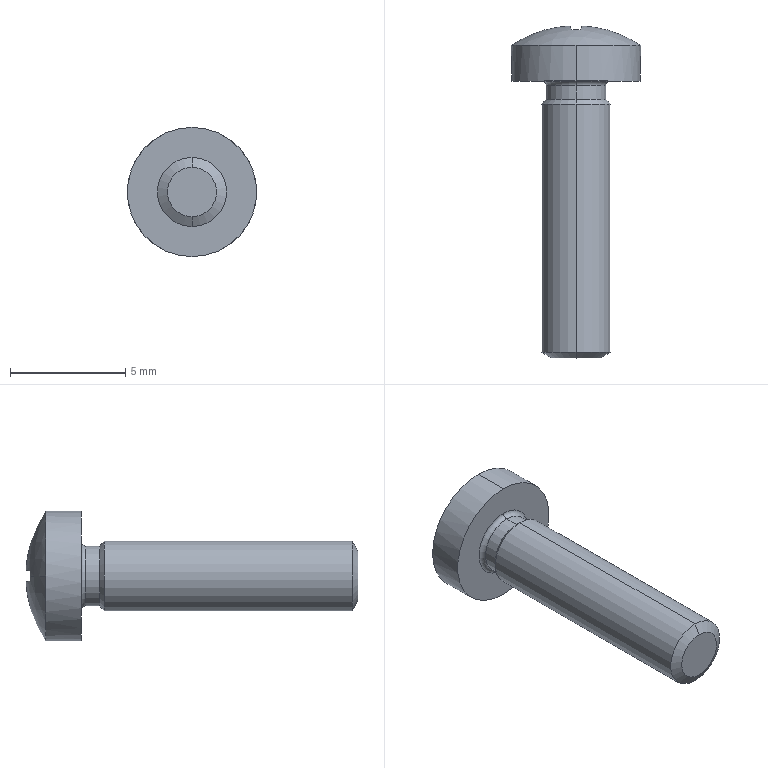Component | SolidWorks | GB_T818-2000PhillipsPanHeadScrewM3_12-3 | 1 solid | 28 faces | box 5.6 x 14.39 x 5.6 mm | volume 130 mm3 | plane 14 | cylinder 6 | cone 4 | torus 2 | sphere 2 | commonest cylinder face diameters 2.598 x2 5.6 x2 3 x2
build123d program:
from build123d import *


with BuildPart() as part:
    # Sketch2 → Base-Revolve (revolve)
    with BuildSketch(Plane.XY, mode=Mode.PRIVATE) as base_revolve_sk:
        with BuildLine():
            Line((0, 0), (14.4, 0))
            Line((14.4, 0), (14.4, 1.5))
            Line((14.4, 1.5), (3.4, 1.5))
            Line((3.4, 1.5), (3.199, 1.299))
            Line((3.199, 1.299), (2.601, 1.299))
            ThreePointArc((2.601, 1.299), (2.459, 1.358), (2.4, 1.5))
            Line((2.4, 1.5), (2.4, 2.8))
            Line((2.4, 2.8), (0.8575, 2.8))
            ThreePointArc((0.8575, 2.8), (0.2192, 1.464), (0, 0))
        make_face()
    revolve(base_revolve_sk.sketch.rotate(Axis((-1.332, 0, 0), (1, 0, 0)), 90), axis=Axis((-1.332, 0, 0), (1, 0, 0)))

    # Sketch3 → Cut-Revolve1 (revolve, cut)
    with BuildSketch(Plane.XY, mode=Mode.PRIVATE) as cut_revolve1_sk:
        Polygon((14.153, 1.5), (14.653, 1.5), (14.4, 1.067), align=None)
    revolve(cut_revolve1_sk.sketch.rotate(Axis((-0.2428, 0, 0), (1, 0, 0)), 90), axis=Axis((-0.2428, 0, 0), (1, 0, 0)), mode=Mode.SUBTRACT)

    # Sketch5 → Cut-Loft1 section 0
    with BuildSketch(Plane(origin=(0, 0, 0), x_dir=(0, 0, -1), z_dir=(1, 0, 0)), mode=Mode.PRIVATE) as cut_loft1_s0:
        with BuildLine():
            Line((0.25, 1.5), (-0.25, 1.5))
            Line((-0.25, 1.5), (-0.25, -1.5))
            Line((-0.25, -1.5), (0.25, -1.5))
            Line((0.25, -1.5), (0.25, 1.5))
        make_face()
    cut_loft1 = loft([Vertex(1.8, 0, 0), cut_loft1_s0.sketch], mode=Mode.SUBTRACT)

    # Mirror1: Cut-Loft1 across plane
    add(cut_loft1.mirror(Plane(origin=(0, 0, 0), x_dir=(0, 0.7071, 0.7071), z_dir=(0, -0.7071, 0.7071))), mode=Mode.SUBTRACT)


solid = part.part

# Placed as in the assembly
solid = solid.moved(Location((-27.344, 162.966, -166.507), (0, 0, -90)))
STEP:
#1=COLOUR_RGB('',0.7922,0.8196,0.9333);
#2=FILL_AREA_STYLE_COLOUR('',#1);
#3=FILL_AREA_STYLE('',(#2));
#4=SURFACE_STYLE_FILL_AREA(#3);
#5=SURFACE_SIDE_STYLE('',(#4));
#6=SURFACE_STYLE_USAGE(.BOTH.,#5);
#7=PRESENTATION_STYLE_ASSIGNMENT((#6));
#8=CARTESIAN_POINT('',(-1.077,5.849,-6.513));
#9=VERTEX_POINT('',#8);
#10=CARTESIAN_POINT('',(-1.077,5.849,-6.597));
#11=VERTEX_POINT('',#10);
#12=CARTESIAN_POINT('',(-1.077,5.849,-6.555));
#13=DIRECTION('',(0.,1.,0.));
#14=DIRECTION('',(0.,0.,1.));
#15=AXIS2_PLACEMENT_3D('',#12,#13,#14);
#16=CIRCLE('',#15,0.04201);
#17=EDGE_CURVE('',#9,#11,#16,.T.);
#18=ORIENTED_EDGE('',*,*,#17,.T.);
#19=CARTESIAN_POINT('',(-1.077,5.859,-6.614));
#20=VERTEX_POINT('',#19);
#21=CARTESIAN_POINT('',(-1.077,5.859,-6.614));
#22=DIRECTION('',(0.,0.4959,-0.8684));
#23=VECTOR('',#22,39.37);
#24=LINE('',#21,#23);
#25=EDGE_CURVE('',#11,#20,#24,.T.);
#26=ORIENTED_EDGE('',*,*,#25,.T.);
#27=CARTESIAN_POINT('',(-1.077,5.859,-6.496));
#28=VERTEX_POINT('',#27);
#29=CARTESIAN_POINT('',(-1.077,5.859,-6.555));
#30=DIRECTION('',(0.,1.,0.));
#31=DIRECTION('',(0.,0.,1.));
#32=AXIS2_PLACEMENT_3D('',#29,#30,#31);
#33=CIRCLE('',#32,0.05906);
#34=EDGE_CURVE('',#28,#20,#33,.T.);
#35=ORIENTED_EDGE('',*,*,#34,.F.);
#36=CARTESIAN_POINT('',(-1.077,5.859,-6.496));
#37=DIRECTION('',(0.,0.4959,0.8684));
#38=VECTOR('',#37,39.37);
#39=LINE('',#36,#38);
#40=EDGE_CURVE('',#9,#28,#39,.T.);
#41=ORIENTED_EDGE('',*,*,#40,.F.);
#42=EDGE_LOOP('',(#18,#26,#35,#41));
#43=FACE_OUTER_BOUND('',#42,.T.);
#44=CARTESIAN_POINT('',(-1.077,5.859,-6.555));
#45=DIRECTION('',(0.,1.,0.));
#46=DIRECTION('',(0.,0.,1.));
#47=AXIS2_PLACEMENT_3D('',#44,#45,#46);
#48=CONICAL_SURFACE('',#47,0.05906,1.052);
#49=ADVANCED_FACE('',(#43),#48,.T.);
#50=CARTESIAN_POINT('',(-1.077,6.29,-6.504));
#51=VERTEX_POINT('',#50);
#52=CARTESIAN_POINT('',(-1.077,6.29,-6.607));
#53=VERTEX_POINT('',#52);
#54=CARTESIAN_POINT('',(-1.077,6.29,-6.555));
#55=DIRECTION('',(0.,1.,0.));
#56=DIRECTION('',(0.,0.,1.));
#57=AXIS2_PLACEMENT_3D('',#54,#55,#56);
#58=CIRCLE('',#57,0.05114);
#59=EDGE_CURVE('',#51,#53,#58,.T.);
#60=ORIENTED_EDGE('',*,*,#59,.F.);
#61=CARTESIAN_POINT('',(-1.077,6.282,-6.496));
#62=VERTEX_POINT('',#61);
#63=CARTESIAN_POINT('',(-1.077,6.282,-6.496));
#64=DIRECTION('',(0.,-0.7071,0.7071));
#65=VECTOR('',#64,39.37);
#66=LINE('',#63,#65);
#67=EDGE_CURVE('',#51,#62,#66,.T.);
#68=ORIENTED_EDGE('',*,*,#67,.T.);
#69=CARTESIAN_POINT('',(-1.077,6.282,-6.614));
#70=VERTEX_POINT('',#69);
#71=CARTESIAN_POINT('',(-1.077,6.282,-6.555));
#72=DIRECTION('',(0.,1.,0.));
#73=DIRECTION('',(0.,0.,1.));
#74=AXIS2_PLACEMENT_3D('',#71,#72,#73);
#75=CIRCLE('',#74,0.05906);
#76=EDGE_CURVE('',#62,#70,#75,.T.);
#77=ORIENTED_EDGE('',*,*,#76,.T.);
#78=CARTESIAN_POINT('',(-1.077,6.282,-6.614));
#79=DIRECTION('',(0.,-0.7071,-0.7071));
#80=VECTOR('',#79,39.37);
#81=LINE('',#78,#80);
#82=EDGE_CURVE('',#53,#70,#81,.T.);
#83=ORIENTED_EDGE('',*,*,#82,.F.);
#84=EDGE_LOOP('',(#60,#68,#77,#83));
#85=FACE_OUTER_BOUND('',#84,.T.);
#86=CARTESIAN_POINT('',(-1.077,6.282,-6.555));
#87=DIRECTION('',(0.,-1.,0.));
#88=DIRECTION('',(0.,0.,-1.));
#89=AXIS2_PLACEMENT_3D('',#86,#87,#88);
#90=CONICAL_SURFACE('',#89,0.05906,0.7854);
#91=ADVANCED_FACE('',(#85),#90,.T.);
#92=ORIENTED_EDGE('',*,*,#59,.T.);
#93=CARTESIAN_POINT('',(-1.077,6.314,-6.607));
#94=VERTEX_POINT('',#93);
#95=CARTESIAN_POINT('',(-1.077,6.468,-6.607));
#96=DIRECTION('',(0.,1.,0.));
#97=VECTOR('',#96,39.37);
#98=LINE('',#95,#97);
#99=EDGE_CURVE('',#53,#94,#98,.T.);
#100=ORIENTED_EDGE('',*,*,#99,.T.);
#101=CARTESIAN_POINT('',(-1.077,6.314,-6.504));
#102=VERTEX_POINT('',#101);
#103=CARTESIAN_POINT('',(-1.077,6.314,-6.555));
#104=DIRECTION('',(0.,1.,0.));
#105=DIRECTION('',(0.,0.,1.));
#106=AXIS2_PLACEMENT_3D('',#103,#104,#105);
#107=CIRCLE('',#106,0.05114);
#108=EDGE_CURVE('',#102,#94,#107,.T.);
#109=ORIENTED_EDGE('',*,*,#108,.F.);
#110=CARTESIAN_POINT('',(-1.077,6.468,-6.504));
#111=DIRECTION('',(0.,1.,0.));
#112=VECTOR('',#111,39.37);
#113=LINE('',#110,#112);
#114=EDGE_CURVE('',#51,#102,#113,.T.);
#115=ORIENTED_EDGE('',*,*,#114,.F.);
#116=EDGE_LOOP('',(#92,#100,#109,#115));
#117=FACE_OUTER_BOUND('',#116,.T.);
#118=CARTESIAN_POINT('',(-1.077,6.468,-6.555));
#119=DIRECTION('',(0.,1.,0.));
#120=DIRECTION('',(0.,0.,1.));
#121=AXIS2_PLACEMENT_3D('',#118,#119,#120);
#122=CYLINDRICAL_SURFACE('',#121,0.05114);
#123=ADVANCED_FACE('',(#117),#122,.T.);
#124=CARTESIAN_POINT('',(-1.077,6.321,-6.614));
#125=VERTEX_POINT('',#124);
#126=CARTESIAN_POINT('',(-1.077,6.321,-6.496));
#127=VERTEX_POINT('',#126);
#128=CARTESIAN_POINT('',(-1.077,6.321,-6.555));
#129=DIRECTION('',(0.,1.,0.));
#130=DIRECTION('',(0.,0.,1.));
#131=AXIS2_PLACEMENT_3D('',#128,#129,#130);
#132=CIRCLE('',#131,0.05906);
#133=EDGE_CURVE('',#125,#127,#132,.T.);
#134=ORIENTED_EDGE('',*,*,#133,.F.);
#135=CARTESIAN_POINT('',(-1.077,6.314,-6.614));
#136=DIRECTION('',(1.,0.,0.));
#137=DIRECTION('',(0.,0.,-1.));
#138=AXIS2_PLACEMENT_3D('',#135,#136,#137);
#139=CIRCLE('',#138,0.007913);
#140=EDGE_CURVE('',#125,#94,#139,.T.);
#141=ORIENTED_EDGE('',*,*,#140,.T.);
#142=CARTESIAN_POINT('',(-1.077,6.314,-6.555));
#143=DIRECTION('',(0.,1.,0.));
#144=DIRECTION('',(0.,0.,1.));
#145=AXIS2_PLACEMENT_3D('',#142,#143,#144);
#146=CIRCLE('',#145,0.05114);
#147=EDGE_CURVE('',#94,#102,#146,.T.);
#148=ORIENTED_EDGE('',*,*,#147,.T.);
#149=CARTESIAN_POINT('',(-1.077,6.314,-6.496));
#150=DIRECTION('',(-1.,0.,0.));
#151=DIRECTION('',(0.,0.,1.));
#152=AXIS2_PLACEMENT_3D('',#149,#150,#151);
#153=CIRCLE('',#152,0.007913);
#154=EDGE_CURVE('',#127,#102,#153,.T.);
#155=ORIENTED_EDGE('',*,*,#154,.F.);
#156=EDGE_LOOP('',(#134,#141,#148,#155));
#157=FACE_OUTER_BOUND('',#156,.T.);
#158=CARTESIAN_POINT('',(-1.077,6.314,-6.555));
#159=DIRECTION('',(0.,1.,0.));
#160=DIRECTION('',(0.,0.,1.));
#161=AXIS2_PLACEMENT_3D('',#158,#159,#160);
#162=TOROIDAL_SURFACE('',#161,0.05906,0.007913);
#163=ADVANCED_FACE('',(#157),#162,.F.);
#164=CARTESIAN_POINT('',(-1.077,6.321,-6.445));
#165=VERTEX_POINT('',#164);
#166=CARTESIAN_POINT('',(-1.077,6.321,-6.666));
#167=VERTEX_POINT('',#166);
#168=CARTESIAN_POINT('',(-1.077,6.321,-6.555));
#169=DIRECTION('',(0.,1.,0.));
#170=DIRECTION('',(0.,0.,1.));
#171=AXIS2_PLACEMENT_3D('',#168,#169,#170);
#172=CIRCLE('',#171,0.1102);
#173=EDGE_CURVE('',#165,#167,#172,.T.);
#174=ORIENTED_EDGE('',*,*,#173,.T.);
#175=CARTESIAN_POINT('',(-1.077,6.382,-6.666));
#176=VERTEX_POINT('',#175);
#177=CARTESIAN_POINT('',(-1.077,6.468,-6.666));
#178=DIRECTION('',(0.,1.,0.));
#179=VECTOR('',#178,39.37);
#180=LINE('',#177,#179);
#181=EDGE_CURVE('',#167,#176,#180,.T.);
#182=ORIENTED_EDGE('',*,*,#181,.T.);
#183=CARTESIAN_POINT('',(-0.9663,6.382,-6.555));
#184=VERTEX_POINT('',#183);
#185=CARTESIAN_POINT('',(-1.077,6.382,-6.555));
#186=DIRECTION('',(0.,1.,0.));
#187=DIRECTION('',(0.,0.,1.));
#188=AXIS2_PLACEMENT_3D('',#185,#186,#187);
#189=CIRCLE('',#188,0.1102);
#190=EDGE_CURVE('',#184,#176,#189,.T.);
#191=ORIENTED_EDGE('',*,*,#190,.F.);
#192=CARTESIAN_POINT('',(-1.077,6.382,-6.445));
#193=VERTEX_POINT('',#192);
#194=CARTESIAN_POINT('',(-1.077,6.382,-6.555));
#195=DIRECTION('',(0.,1.,0.));
#196=DIRECTION('',(0.,0.,1.));
#197=AXIS2_PLACEMENT_3D('',#194,#195,#196);
#198=CIRCLE('',#197,0.1102);
#199=EDGE_CURVE('',#193,#184,#198,.T.);
#200=ORIENTED_EDGE('',*,*,#199,.F.);
#201=CARTESIAN_POINT('',(-1.077,6.468,-6.445));
#202=DIRECTION('',(0.,1.,0.));
#203=VECTOR('',#202,39.37);
#204=LINE('',#201,#203);
#205=EDGE_CURVE('',#165,#193,#204,.T.);
#206=ORIENTED_EDGE('',*,*,#205,.F.);
#207=EDGE_LOOP('',(#174,#182,#191,#200,#206));
#208=FACE_OUTER_BOUND('',#207,.T.);
#209=CARTESIAN_POINT('',(-1.077,6.468,-6.555));
#210=DIRECTION('',(0.,1.,0.));
#211=DIRECTION('',(0.,0.,1.));
#212=AXIS2_PLACEMENT_3D('',#209,#210,#211);
#213=CYLINDRICAL_SURFACE('',#212,0.1102);
#214=ADVANCED_FACE('',(#208),#213,.T.);
#215=ORIENTED_EDGE('',*,*,#190,.T.);
#216=CARTESIAN_POINT('',(-1.187,6.382,-6.555));
#217=VERTEX_POINT('',#216);
#218=CARTESIAN_POINT('',(-1.077,6.382,-6.555));
#219=DIRECTION('',(0.,1.,0.));
#220=DIRECTION('',(0.,0.,1.));
#221=AXIS2_PLACEMENT_3D('',#218,#219,#220);
#222=CIRCLE('',#221,0.1102);
#223=EDGE_CURVE('',#176,#217,#222,.T.);
#224=ORIENTED_EDGE('',*,*,#223,.T.);
#225=CARTESIAN_POINT('',(-1.13,6.409,-6.555));
#226=VERTEX_POINT('',#225);
#227=CARTESIAN_POINT('',(-1.077,6.219,-6.555));
#228=DIRECTION('',(0.,0.,-1.));
#229=DIRECTION('',(-1.,0.,0.));
#230=AXIS2_PLACEMENT_3D('',#227,#228,#229);
#231=CIRCLE('',#230,0.1969);
#232=EDGE_CURVE('',#217,#226,#231,.T.);
#233=ORIENTED_EDGE('',*,*,#232,.T.);
#234=CARTESIAN_POINT('',(-1.129,6.409,-6.564));
#235=VERTEX_POINT('',#234);
#236=CARTESIAN_POINT('',(-1.015,6.271,-6.555));
#237=DIRECTION('',(-0.7682,-0.6402,0.));
#238=DIRECTION('',(0.6402,-0.7682,0.));
#239=AXIS2_PLACEMENT_3D('',#236,#237,#238);
#240=CIRCLE('',#239,0.1796);
#241=EDGE_CURVE('',#226,#235,#240,.T.);
#242=ORIENTED_EDGE('',*,*,#241,.T.);
#243=CARTESIAN_POINT('',(-1.086,6.415,-6.565));
#244=VERTEX_POINT('',#243);
#245=CARTESIAN_POINT('',(-1.077,6.222,-6.538));
#246=DIRECTION('',(0.,-0.1376,-0.9905));
#247=DIRECTION('',(0.,0.9905,-0.1376));
#248=AXIS2_PLACEMENT_3D('',#245,#246,#247);
#249=CIRCLE('',#248,0.1961);
#250=EDGE_CURVE('',#235,#244,#249,.T.);
#251=ORIENTED_EDGE('',*,*,#250,.T.);
#252=CARTESIAN_POINT('',(-1.085,6.409,-6.608));
#253=VERTEX_POINT('',#252);
#254=CARTESIAN_POINT('',(-1.059,6.222,-6.555));
#255=DIRECTION('',(-0.9905,-0.1376,-0.));
#256=DIRECTION('',(0.1376,-0.9905,0.));
#257=AXIS2_PLACEMENT_3D('',#254,#255,#256);
#258=CIRCLE('',#257,0.1961);
#259=EDGE_CURVE('',#244,#253,#258,.T.);
#260=ORIENTED_EDGE('',*,*,#259,.T.);
#261=CARTESIAN_POINT('',(-1.068,6.409,-6.608));
#262=VERTEX_POINT('',#261);
#263=CARTESIAN_POINT('',(-1.077,6.271,-6.493));
#264=DIRECTION('',(0.,-0.6402,-0.7682));
#265=DIRECTION('',(0.,0.7682,-0.6402));
#266=AXIS2_PLACEMENT_3D('',#263,#264,#265);
#267=CIRCLE('',#266,0.1796);
#268=EDGE_CURVE('',#253,#262,#267,.T.);
#269=ORIENTED_EDGE('',*,*,#268,.T.);
#270=CARTESIAN_POINT('',(-1.067,6.415,-6.565));
#271=VERTEX_POINT('',#270);
#272=CARTESIAN_POINT('',(-1.094,6.222,-6.555));
#273=DIRECTION('',(0.9905,-0.1376,0.));
#274=DIRECTION('',(0.1376,0.9905,0.));
#275=AXIS2_PLACEMENT_3D('',#272,#273,#274);
#276=CIRCLE('',#275,0.1961);
#277=EDGE_CURVE('',#262,#271,#276,.T.);
#278=ORIENTED_EDGE('',*,*,#277,.T.);
#279=CARTESIAN_POINT('',(-1.024,6.409,-6.564));
#280=VERTEX_POINT('',#279);
#281=CARTESIAN_POINT('',(-1.077,6.222,-6.538));
#282=DIRECTION('',(0.,-0.1376,-0.9905));
#283=DIRECTION('',(0.,0.9905,-0.1376));
#284=AXIS2_PLACEMENT_3D('',#281,#282,#283);
#285=CIRCLE('',#284,0.1961);
#286=EDGE_CURVE('',#271,#280,#285,.T.);
#287=ORIENTED_EDGE('',*,*,#286,.T.);
#288=CARTESIAN_POINT('',(-1.024,6.409,-6.555));
#289=VERTEX_POINT('',#288);
#290=CARTESIAN_POINT('',(-1.139,6.271,-6.555));
#291=DIRECTION('',(0.7682,-0.6402,0.));
#292=DIRECTION('',(0.6402,0.7682,0.));
#293=AXIS2_PLACEMENT_3D('',#290,#291,#292);
#294=CIRCLE('',#293,0.1796);
#295=EDGE_CURVE('',#280,#289,#294,.T.);
#296=ORIENTED_EDGE('',*,*,#295,.T.);
#297=CARTESIAN_POINT('',(-1.077,6.219,-6.555));
#298=DIRECTION('',(0.,0.,1.));
#299=DIRECTION('',(1.,0.,0.));
#300=AXIS2_PLACEMENT_3D('',#297,#298,#299);
#301=CIRCLE('',#300,0.1969);
#302=EDGE_CURVE('',#184,#289,#301,.T.);
#303=ORIENTED_EDGE('',*,*,#302,.F.);
#304=EDGE_LOOP('',(#215,#224,#233,#242,#251,#260,#269,#278,#287,#296,#303));
#305=FACE_OUTER_BOUND('',#304,.T.);
#306=CARTESIAN_POINT('',(-1.077,6.219,-6.555));
#307=DIRECTION('',(0.,0.,-1.));
#308=DIRECTION('',(1.,0.,0.));
#309=AXIS2_PLACEMENT_3D('',#306,#307,#308);
#310=SPHERICAL_SURFACE('',#309,0.1969);
#311=ADVANCED_FACE('',(#305),#310,.T.);
#312=ORIENTED_EDGE('',*,*,#34,.T.);
#313=CARTESIAN_POINT('',(-1.077,6.468,-6.614));
#314=DIRECTION('',(0.,1.,0.));
#315=VECTOR('',#314,39.37);
#316=LINE('',#313,#315);
#317=EDGE_CURVE('',#20,#70,#316,.T.);
#318=ORIENTED_EDGE('',*,*,#317,.T.);
#319=ORIENTED_EDGE('',*,*,#76,.F.);
#320=CARTESIAN_POINT('',(-1.077,6.468,-6.496));
#321=DIRECTION('',(0.,1.,0.));
#322=VECTOR('',#321,39.37);
#323=LINE('',#320,#322);
#324=EDGE_CURVE('',#28,#62,#323,.T.);
#325=ORIENTED_EDGE('',*,*,#324,.F.);
#326=EDGE_LOOP('',(#312,#318,#319,#325));
#327=FACE_OUTER_BOUND('',#326,.T.);
#328=CARTESIAN_POINT('',(-1.077,6.468,-6.555));
#329=DIRECTION('',(0.,1.,0.));
#330=DIRECTION('',(0.,0.,1.));
#331=AXIS2_PLACEMENT_3D('',#328,#329,#330);
#332=CYLINDRICAL_SURFACE('',#331,0.05906);
#333=ADVANCED_FACE('',(#327),#332,.T.);
#334=CARTESIAN_POINT('',(-1.077,6.345,-6.555));
#335=VERTEX_POINT('',#334);
#336=CARTESIAN_POINT('',(-1.077,6.345,-6.555));
#337=DIRECTION('',(-0.6366,0.7639,-0.1061));
#338=VECTOR('',#337,39.37);
#339=LINE('',#336,#338);
#340=EDGE_CURVE('',#335,#235,#339,.T.);
#341=ORIENTED_EDGE('',*,*,#340,.F.);
#342=CARTESIAN_POINT('',(-1.077,6.345,-6.555));
#343=DIRECTION('',(-0.1363,0.9813,-0.1363));
#344=VECTOR('',#343,39.37);
#345=LINE('',#342,#344);
#346=EDGE_CURVE('',#335,#244,#345,.T.);
#347=ORIENTED_EDGE('',*,*,#346,.T.);
#348=ORIENTED_EDGE('',*,*,#250,.F.);
#349=EDGE_LOOP('',(#341,#347,#348));
#350=FACE_OUTER_BOUND('',#349,.T.);
#351=CARTESIAN_POINT('',(-1.077,6.345,-6.555));
#352=DIRECTION('',(0.,-0.1376,-0.9905));
#353=DIRECTION('',(0.,0.9905,-0.1376));
#354=AXIS2_PLACEMENT_3D('',#351,#352,#353);
#355=PLANE('',#354);
#356=ADVANCED_FACE('',(#350),#355,.F.);
#357=CARTESIAN_POINT('',(-1.086,6.415,-6.546));
#358=VERTEX_POINT('',#357);
#359=CARTESIAN_POINT('',(-1.129,6.409,-6.547));
#360=VERTEX_POINT('',#359);
#361=CARTESIAN_POINT('',(-1.077,6.222,-6.573));
#362=DIRECTION('',(0.,-0.1376,0.9905));
#363=DIRECTION('',(0.,-0.9905,-0.1376));
#364=AXIS2_PLACEMENT_3D('',#361,#362,#363);
#365=CIRCLE('',#364,0.1961);
#366=EDGE_CURVE('',#358,#360,#365,.T.);
#367=ORIENTED_EDGE('',*,*,#366,.F.);
#368=CARTESIAN_POINT('',(-1.077,6.345,-6.555));
#369=DIRECTION('',(0.1363,-0.9813,-0.1363));
#370=VECTOR('',#369,39.37);
#371=LINE('',#368,#370);
#372=EDGE_CURVE('',#358,#335,#371,.T.);
#373=ORIENTED_EDGE('',*,*,#372,.T.);
#374=CARTESIAN_POINT('',(-1.077,6.345,-6.555));
#375=DIRECTION('',(-0.6366,0.7639,0.1061));
#376=VECTOR('',#375,39.37);
#377=LINE('',#374,#376);
#378=EDGE_CURVE('',#335,#360,#377,.T.);
#379=ORIENTED_EDGE('',*,*,#378,.T.);
#380=EDGE_LOOP('',(#367,#373,#379));
#381=FACE_OUTER_BOUND('',#380,.T.);
#382=CARTESIAN_POINT('',(-1.077,6.345,-6.555));
#383=DIRECTION('',(0.,-0.1376,0.9905));
#384=DIRECTION('',(0.,-0.9905,-0.1376));
#385=AXIS2_PLACEMENT_3D('',#382,#383,#384);
#386=PLANE('',#385);
#387=ADVANCED_FACE('',(#381),#386,.F.);
#388=ORIENTED_EDGE('',*,*,#317,.F.);
#389=CARTESIAN_POINT('',(-1.077,5.859,-6.555));
#390=DIRECTION('',(0.,1.,0.));
#391=DIRECTION('',(0.,0.,1.));
#392=AXIS2_PLACEMENT_3D('',#389,#390,#391);
#393=CIRCLE('',#392,0.05906);
#394=EDGE_CURVE('',#20,#28,#393,.T.);
#395=ORIENTED_EDGE('',*,*,#394,.T.);
#396=ORIENTED_EDGE('',*,*,#324,.T.);
#397=CARTESIAN_POINT('',(-1.077,6.282,-6.555));
#398=DIRECTION('',(0.,1.,0.));
#399=DIRECTION('',(0.,0.,1.));
#400=AXIS2_PLACEMENT_3D('',#397,#398,#399);
#401=CIRCLE('',#400,0.05906);
#402=EDGE_CURVE('',#70,#62,#401,.T.);
#403=ORIENTED_EDGE('',*,*,#402,.F.);
#404=EDGE_LOOP('',(#388,#395,#396,#403));
#405=FACE_OUTER_BOUND('',#404,.T.);
#406=CARTESIAN_POINT('',(-1.077,6.468,-6.555));
#407=DIRECTION('',(0.,1.,0.));
#408=DIRECTION('',(0.,0.,1.));
#409=AXIS2_PLACEMENT_3D('',#406,#407,#408);
#410=CYLINDRICAL_SURFACE('',#409,0.05906);
#411=ADVANCED_FACE('',(#405),#410,.T.);
#412=ORIENTED_EDGE('',*,*,#232,.F.);
#413=CARTESIAN_POINT('',(-1.077,6.382,-6.555));
#414=DIRECTION('',(0.,1.,0.));
#415=DIRECTION('',(0.,0.,1.));
#416=AXIS2_PLACEMENT_3D('',#413,#414,#415);
#417=CIRCLE('',#416,0.1102);
#418=EDGE_CURVE('',#217,#193,#417,.T.);
#419=ORIENTED_EDGE('',*,*,#418,.T.);
#420=ORIENTED_EDGE('',*,*,#199,.T.);
#421=ORIENTED_EDGE('',*,*,#302,.T.);
#422=CARTESIAN_POINT('',(-1.024,6.409,-6.547));
#423=VERTEX_POINT('',#422);
#424=CARTESIAN_POINT('',(-1.139,6.271,-6.555));
#425=DIRECTION('',(0.7682,-0.6402,0.));
#426=DIRECTION('',(0.6402,0.7682,0.));
#427=AXIS2_PLACEMENT_3D('',#424,#425,#426);
#428=CIRCLE('',#427,0.1796);
#429=EDGE_CURVE('',#289,#423,#428,.T.);
#430=ORIENTED_EDGE('',*,*,#429,.T.);
#431=CARTESIAN_POINT('',(-1.067,6.415,-6.546));
#432=VERTEX_POINT('',#431);
#433=CARTESIAN_POINT('',(-1.077,6.222,-6.573));
#434=DIRECTION('',(0.,-0.1376,0.9905));
#435=DIRECTION('',(0.,-0.9905,-0.1376));
#436=AXIS2_PLACEMENT_3D('',#433,#434,#435);
#437=CIRCLE('',#436,0.1961);
#438=EDGE_CURVE('',#423,#432,#437,.T.);
#439=ORIENTED_EDGE('',*,*,#438,.T.);
#440=CARTESIAN_POINT('',(-1.068,6.409,-6.503));
#441=VERTEX_POINT('',#440);
#442=CARTESIAN_POINT('',(-1.094,6.222,-6.555));
#443=DIRECTION('',(0.9905,-0.1376,0.));
#444=DIRECTION('',(0.1376,0.9905,0.));
#445=AXIS2_PLACEMENT_3D('',#442,#443,#444);
#446=CIRCLE('',#445,0.1961);
#447=EDGE_CURVE('',#432,#441,#446,.T.);
#448=ORIENTED_EDGE('',*,*,#447,.T.);
#449=CARTESIAN_POINT('',(-1.085,6.409,-6.503));
#450=VERTEX_POINT('',#449);
#451=CARTESIAN_POINT('',(-1.077,6.271,-6.617));
#452=DIRECTION('',(-0.,-0.6402,0.7682));
#453=DIRECTION('',(0.,-0.7682,-0.6402));
#454=AXIS2_PLACEMENT_3D('',#451,#452,#453);
#455=CIRCLE('',#454,0.1796);
#456=EDGE_CURVE('',#441,#450,#455,.T.);
#457=ORIENTED_EDGE('',*,*,#456,.T.);
#458=CARTESIAN_POINT('',(-1.059,6.222,-6.555));
#459=DIRECTION('',(-0.9905,-0.1376,-0.));
#460=DIRECTION('',(0.1376,-0.9905,0.));
#461=AXIS2_PLACEMENT_3D('',#458,#459,#460);
#462=CIRCLE('',#461,0.1961);
#463=EDGE_CURVE('',#450,#358,#462,.T.);
#464=ORIENTED_EDGE('',*,*,#463,.T.);
#465=ORIENTED_EDGE('',*,*,#366,.T.);
#466=CARTESIAN_POINT('',(-1.015,6.271,-6.555));
#467=DIRECTION('',(-0.7682,-0.6402,0.));
#468=DIRECTION('',(0.6402,-0.7682,0.));
#469=AXIS2_PLACEMENT_3D('',#466,#467,#468);
#470=CIRCLE('',#469,0.1796);
#471=EDGE_CURVE('',#360,#226,#470,.T.);
#472=ORIENTED_EDGE('',*,*,#471,.T.);
#473=EDGE_LOOP('',(#412,#419,#420,#421,#430,#439,#448,#457,#464,#465,#472));
#474=FACE_OUTER_BOUND('',#473,.T.);
#475=CARTESIAN_POINT('',(-1.077,6.219,-6.555));
#476=DIRECTION('',(0.,0.,-1.));
#477=DIRECTION('',(1.,0.,0.));
#478=AXIS2_PLACEMENT_3D('',#475,#476,#477);
#479=SPHERICAL_SURFACE('',#478,0.1969);
#480=ADVANCED_FACE('',(#474),#479,.T.);
#481=ORIENTED_EDGE('',*,*,#181,.F.);
#482=CARTESIAN_POINT('',(-1.077,6.321,-6.555));
#483=DIRECTION('',(0.,1.,0.));
#484=DIRECTION('',(0.,0.,1.));
#485=AXIS2_PLACEMENT_3D('',#482,#483,#484);
#486=CIRCLE('',#485,0.1102);
#487=EDGE_CURVE('',#167,#165,#486,.T.);
#488=ORIENTED_EDGE('',*,*,#487,.T.);
#489=ORIENTED_EDGE('',*,*,#205,.T.);
#490=ORIENTED_EDGE('',*,*,#418,.F.);
#491=ORIENTED_EDGE('',*,*,#223,.F.);
#492=EDGE_LOOP('',(#481,#488,#489,#490,#491));
#493=FACE_OUTER_BOUND('',#492,.T.);
#494=CARTESIAN_POINT('',(-1.077,6.468,-6.555));
#495=DIRECTION('',(0.,1.,0.));
#496=DIRECTION('',(0.,0.,1.));
#497=AXIS2_PLACEMENT_3D('',#494,#495,#496);
#498=CYLINDRICAL_SURFACE('',#497,0.1102);
#499=ADVANCED_FACE('',(#493),#498,.T.);
#500=ORIENTED_EDGE('',*,*,#173,.F.);
#501=ORIENTED_EDGE('',*,*,#487,.F.);
#502=EDGE_LOOP('',(#500,#501));
#503=FACE_OUTER_BOUND('',#502,.T.);
#504=CARTESIAN_POINT('',(-1.077,6.321,-6.555));
#505=DIRECTION('',(0.,1.,0.));
#506=DIRECTION('',(0.,0.,1.));
#507=AXIS2_PLACEMENT_3D('',#504,#505,#506);
#508=CIRCLE('',#507,0.05906);
#509=EDGE_CURVE('',#127,#125,#508,.T.);
#510=ORIENTED_EDGE('',*,*,#509,.T.);
#511=ORIENTED_EDGE('',*,*,#133,.T.);
#512=EDGE_LOOP('',(#510,#511));
#513=FACE_BOUND('',#512,.T.);
#514=CARTESIAN_POINT('',(-1.017,6.321,-6.555));
#515=DIRECTION('',(0.,1.,0.));
#516=DIRECTION('',(0.,0.,1.));
#517=AXIS2_PLACEMENT_3D('',#514,#515,#516);
#518=PLANE('',#517);
#519=ADVANCED_FACE('',(#503,#513),#518,.F.);
#520=ORIENTED_EDGE('',*,*,#140,.F.);
#521=ORIENTED_EDGE('',*,*,#509,.F.);
#522=ORIENTED_EDGE('',*,*,#154,.T.);
#523=ORIENTED_EDGE('',*,*,#108,.T.);
#524=EDGE_LOOP('',(#520,#521,#522,#523));
#525=FACE_OUTER_BOUND('',#524,.T.);
#526=CARTESIAN_POINT('',(-1.077,6.314,-6.555));
#527=DIRECTION('',(0.,1.,0.));
#528=DIRECTION('',(0.,0.,1.));
#529=AXIS2_PLACEMENT_3D('',#526,#527,#528);
#530=TOROIDAL_SURFACE('',#529,0.05906,0.007913);
#531=ADVANCED_FACE('',(#525),#530,.F.);
#532=ORIENTED_EDGE('',*,*,#99,.F.);
#533=CARTESIAN_POINT('',(-1.077,6.29,-6.555));
#534=DIRECTION('',(0.,1.,0.));
#535=DIRECTION('',(0.,0.,1.));
#536=AXIS2_PLACEMENT_3D('',#533,#534,#535);
#537=CIRCLE('',#536,0.05114);
#538=EDGE_CURVE('',#53,#51,#537,.T.);
#539=ORIENTED_EDGE('',*,*,#538,.T.);
#540=ORIENTED_EDGE('',*,*,#114,.T.);
#541=ORIENTED_EDGE('',*,*,#147,.F.);
#542=EDGE_LOOP('',(#532,#539,#540,#541));
#543=FACE_OUTER_BOUND('',#542,.T.);
#544=CARTESIAN_POINT('',(-1.077,6.468,-6.555));
#545=DIRECTION('',(0.,1.,0.));
#546=DIRECTION('',(0.,0.,1.));
#547=AXIS2_PLACEMENT_3D('',#544,#545,#546);
#548=CYLINDRICAL_SURFACE('',#547,0.05114);
#549=ADVANCED_FACE('',(#543),#548,.T.);
#550=ORIENTED_EDGE('',*,*,#67,.F.);
#551=ORIENTED_EDGE('',*,*,#538,.F.);
#552=ORIENTED_EDGE('',*,*,#82,.T.);
#553=ORIENTED_EDGE('',*,*,#402,.T.);
#554=EDGE_LOOP('',(#550,#551,#552,#553));
#555=FACE_OUTER_BOUND('',#554,.T.);
#556=CARTESIAN_POINT('',(-1.077,6.282,-6.555));
#557=DIRECTION('',(0.,-1.,0.));
#558=DIRECTION('',(0.,0.,-1.));
#559=AXIS2_PLACEMENT_3D('',#556,#557,#558);
#560=CONICAL_SURFACE('',#559,0.05906,0.7854);
#561=ADVANCED_FACE('',(#555),#560,.T.);
#562=ORIENTED_EDGE('',*,*,#25,.F.);
#563=CARTESIAN_POINT('',(-1.077,5.849,-6.555));
#564=DIRECTION('',(0.,1.,0.));
#565=DIRECTION('',(0.,0.,1.));
#566=AXIS2_PLACEMENT_3D('',#563,#564,#565);
#567=CIRCLE('',#566,0.04201);
#568=EDGE_CURVE('',#11,#9,#567,.T.);
#569=ORIENTED_EDGE('',*,*,#568,.T.);
#570=ORIENTED_EDGE('',*,*,#40,.T.);
#571=ORIENTED_EDGE('',*,*,#394,.F.);
#572=EDGE_LOOP('',(#562,#569,#570,#571));
#573=FACE_OUTER_BOUND('',#572,.T.);
#574=CARTESIAN_POINT('',(-1.077,5.859,-6.555));
#575=DIRECTION('',(0.,1.,0.));
#576=DIRECTION('',(0.,0.,1.));
#577=AXIS2_PLACEMENT_3D('',#574,#575,#576);
#578=CONICAL_SURFACE('',#577,0.05906,1.052);
#579=ADVANCED_FACE('',(#573),#578,.T.);
#580=ORIENTED_EDGE('',*,*,#17,.F.);
#581=ORIENTED_EDGE('',*,*,#568,.F.);
#582=EDGE_LOOP('',(#580,#581));
#583=FACE_OUTER_BOUND('',#582,.T.);
#584=CARTESIAN_POINT('',(-1.077,5.849,-6.555));
#585=DIRECTION('',(0.,1.,0.));
#586=DIRECTION('',(0.,0.,1.));
#587=AXIS2_PLACEMENT_3D('',#584,#585,#586);
#588=PLANE('',#587);
#589=ADVANCED_FACE('',(#583),#588,.F.);
#590=ORIENTED_EDGE('',*,*,#286,.F.);
#591=CARTESIAN_POINT('',(-1.077,6.345,-6.555));
#592=DIRECTION('',(-0.1363,-0.9813,0.1363));
#593=VECTOR('',#592,39.37);
#594=LINE('',#591,#593);
#595=EDGE_CURVE('',#271,#335,#594,.T.);
#596=ORIENTED_EDGE('',*,*,#595,.T.);
#597=CARTESIAN_POINT('',(-1.077,6.345,-6.555));
#598=DIRECTION('',(0.6366,0.7639,-0.1061));
#599=VECTOR('',#598,39.37);
#600=LINE('',#597,#599);
#601=EDGE_CURVE('',#335,#280,#600,.T.);
#602=ORIENTED_EDGE('',*,*,#601,.T.);
#603=EDGE_LOOP('',(#590,#596,#602));
#604=FACE_OUTER_BOUND('',#603,.T.);
#605=CARTESIAN_POINT('',(-1.077,6.345,-6.555));
#606=DIRECTION('',(0.,-0.1376,-0.9905));
#607=DIRECTION('',(0.,0.9905,-0.1376));
#608=AXIS2_PLACEMENT_3D('',#605,#606,#607);
#609=PLANE('',#608);
#610=ADVANCED_FACE('',(#604),#609,.F.);
#611=ORIENTED_EDGE('',*,*,#601,.F.);
#612=CARTESIAN_POINT('',(-1.077,6.345,-6.555));
#613=DIRECTION('',(0.6366,0.7639,0.1061));
#614=VECTOR('',#613,39.37);
#615=LINE('',#612,#614);
#616=EDGE_CURVE('',#335,#423,#615,.T.);
#617=ORIENTED_EDGE('',*,*,#616,.T.);
#618=ORIENTED_EDGE('',*,*,#429,.F.);
#619=ORIENTED_EDGE('',*,*,#295,.F.);
#620=EDGE_LOOP('',(#611,#617,#618,#619));
#621=FACE_OUTER_BOUND('',#620,.T.);
#622=CARTESIAN_POINT('',(-1.017,6.416,-6.565));
#623=DIRECTION('',(0.7682,-0.6402,0.));
#624=DIRECTION('',(0.6402,0.7682,0.));
#625=AXIS2_PLACEMENT_3D('',#622,#623,#624);
#626=PLANE('',#625);
#627=ADVANCED_FACE('',(#621),#626,.F.);
#628=ORIENTED_EDGE('',*,*,#378,.F.);
#629=ORIENTED_EDGE('',*,*,#340,.T.);
#630=ORIENTED_EDGE('',*,*,#241,.F.);
#631=ORIENTED_EDGE('',*,*,#471,.F.);
#632=EDGE_LOOP('',(#628,#629,#630,#631));
#633=FACE_OUTER_BOUND('',#632,.T.);
#634=CARTESIAN_POINT('',(-1.136,6.416,-6.546));
#635=DIRECTION('',(-0.7682,-0.6402,0.));
#636=DIRECTION('',(0.6402,-0.7682,0.));
#637=AXIS2_PLACEMENT_3D('',#634,#635,#636);
#638=PLANE('',#637);
#639=ADVANCED_FACE('',(#633),#638,.F.);
#640=ORIENTED_EDGE('',*,*,#616,.F.);
#641=CARTESIAN_POINT('',(-1.077,6.345,-6.555));
#642=DIRECTION('',(0.1363,0.9813,0.1363));
#643=VECTOR('',#642,39.37);
#644=LINE('',#641,#643);
#645=EDGE_CURVE('',#335,#432,#644,.T.);
#646=ORIENTED_EDGE('',*,*,#645,.T.);
#647=ORIENTED_EDGE('',*,*,#438,.F.);
#648=EDGE_LOOP('',(#640,#646,#647));
#649=FACE_OUTER_BOUND('',#648,.T.);
#650=CARTESIAN_POINT('',(-1.077,6.345,-6.555));
#651=DIRECTION('',(0.,-0.1376,0.9905));
#652=DIRECTION('',(0.,-0.9905,-0.1376));
#653=AXIS2_PLACEMENT_3D('',#650,#651,#652);
#654=PLANE('',#653);
#655=ADVANCED_FACE('',(#649),#654,.F.);
#656=CARTESIAN_POINT('',(-1.077,6.345,-6.555));
#657=DIRECTION('',(-0.1061,0.7639,0.6366));
#658=VECTOR('',#657,39.37);
#659=LINE('',#656,#658);
#660=EDGE_CURVE('',#335,#450,#659,.T.);
#661=ORIENTED_EDGE('',*,*,#660,.F.);
#662=ORIENTED_EDGE('',*,*,#372,.F.);
#663=ORIENTED_EDGE('',*,*,#463,.F.);
#664=EDGE_LOOP('',(#661,#662,#663));
#665=FACE_OUTER_BOUND('',#664,.T.);
#666=CARTESIAN_POINT('',(-1.077,6.345,-6.555));
#667=DIRECTION('',(-0.9905,-0.1376,-0.));
#668=DIRECTION('',(-0.1376,0.9905,-0.));
#669=AXIS2_PLACEMENT_3D('',#666,#667,#668);
#670=PLANE('',#669);
#671=ADVANCED_FACE('',(#665),#670,.F.);
#672=ORIENTED_EDGE('',*,*,#645,.F.);
#673=CARTESIAN_POINT('',(-1.077,6.345,-6.555));
#674=DIRECTION('',(0.1061,0.7639,0.6366));
#675=VECTOR('',#674,39.37);
#676=LINE('',#673,#675);
#677=EDGE_CURVE('',#335,#441,#676,.T.);
#678=ORIENTED_EDGE('',*,*,#677,.T.);
#679=ORIENTED_EDGE('',*,*,#447,.F.);
#680=EDGE_LOOP('',(#672,#678,#679));
#681=FACE_OUTER_BOUND('',#680,.T.);
#682=CARTESIAN_POINT('',(-1.077,6.345,-6.555));
#683=DIRECTION('',(0.9905,-0.1376,0.));
#684=DIRECTION('',(-0.1376,-0.9905,-0.));
#685=AXIS2_PLACEMENT_3D('',#682,#683,#684);
#686=PLANE('',#685);
#687=ADVANCED_FACE('',(#681),#686,.F.);
#688=ORIENTED_EDGE('',*,*,#677,.F.);
#689=ORIENTED_EDGE('',*,*,#660,.T.);
#690=ORIENTED_EDGE('',*,*,#456,.F.);
#691=EDGE_LOOP('',(#688,#689,#690));
#692=FACE_OUTER_BOUND('',#691,.T.);
#693=CARTESIAN_POINT('',(-1.086,6.416,-6.496));
#694=DIRECTION('',(-0.,-0.6402,0.7682));
#695=DIRECTION('',(-0.,0.7682,0.6402));
#696=AXIS2_PLACEMENT_3D('',#693,#694,#695);
#697=PLANE('',#696);
#698=ADVANCED_FACE('',(#692),#697,.F.);
#699=ORIENTED_EDGE('',*,*,#346,.F.);
#700=CARTESIAN_POINT('',(-1.077,6.345,-6.555));
#701=DIRECTION('',(-0.1061,0.7639,-0.6366));
#702=VECTOR('',#701,39.37);
#703=LINE('',#700,#702);
#704=EDGE_CURVE('',#335,#253,#703,.T.);
#705=ORIENTED_EDGE('',*,*,#704,.T.);
#706=ORIENTED_EDGE('',*,*,#259,.F.);
#707=EDGE_LOOP('',(#699,#705,#706));
#708=FACE_OUTER_BOUND('',#707,.T.);
#709=CARTESIAN_POINT('',(-1.077,6.345,-6.555));
#710=DIRECTION('',(-0.9905,-0.1376,-0.));
#711=DIRECTION('',(-0.1376,0.9905,-0.));
#712=AXIS2_PLACEMENT_3D('',#709,#710,#711);
#713=PLANE('',#712);
#714=ADVANCED_FACE('',(#708),#713,.F.);
#715=ORIENTED_EDGE('',*,*,#704,.F.);
#716=CARTESIAN_POINT('',(-1.077,6.345,-6.555));
#717=DIRECTION('',(0.1061,0.7639,-0.6366));
#718=VECTOR('',#717,39.37);
#719=LINE('',#716,#718);
#720=EDGE_CURVE('',#335,#262,#719,.T.);
#721=ORIENTED_EDGE('',*,*,#720,.T.);
#722=ORIENTED_EDGE('',*,*,#268,.F.);
#723=EDGE_LOOP('',(#715,#721,#722));
#724=FACE_OUTER_BOUND('',#723,.T.);
#725=CARTESIAN_POINT('',(-1.067,6.416,-6.614));
#726=DIRECTION('',(0.,-0.6402,-0.7682));
#727=DIRECTION('',(-0.,-0.7682,0.6402));
#728=AXIS2_PLACEMENT_3D('',#725,#726,#727);
#729=PLANE('',#728);
#730=ADVANCED_FACE('',(#724),#729,.F.);
#731=ORIENTED_EDGE('',*,*,#720,.F.);
#732=ORIENTED_EDGE('',*,*,#595,.F.);
#733=ORIENTED_EDGE('',*,*,#277,.F.);
#734=EDGE_LOOP('',(#731,#732,#733));
#735=FACE_OUTER_BOUND('',#734,.T.);
#736=CARTESIAN_POINT('',(-1.077,6.345,-6.555));
#737=DIRECTION('',(0.9905,-0.1376,0.));
#738=DIRECTION('',(-0.1376,-0.9905,-0.));
#739=AXIS2_PLACEMENT_3D('',#736,#737,#738);
#740=PLANE('',#739);
#741=ADVANCED_FACE('',(#735),#740,.F.);
#742=CLOSED_SHELL('',(#49,#91,#123,#163,#214,#311,#333,#356,#387,#411,#480,#499,#519,#531,#549,#561,#579,#589,#610,#627,#639,#655,#671,#687,#698,#714,#730,#741));
#743=MANIFOLD_SOLID_BREP('',#742);
#744=STYLED_ITEM('',(#7),#743);
#745=(LENGTH_UNIT()NAMED_UNIT(*)SI_UNIT($,.METRE.));
#746=LENGTH_MEASURE_WITH_UNIT(LENGTH_MEASURE(0.0254),#745);
#747=DIMENSIONAL_EXPONENTS(1.,0.,0.,0.,0.,0.,0.);
#748=(CONVERSION_BASED_UNIT('',#746)LENGTH_UNIT()NAMED_UNIT(#747));
#749=UNCERTAINTY_MEASURE_WITH_UNIT(LENGTH_MEASURE(0.00001),#748,'','');
#750=(NAMED_UNIT(*)PLANE_ANGLE_UNIT()SI_UNIT($,.RADIAN.));
#751=(NAMED_UNIT(*)SI_UNIT($,.STERADIAN.)SOLID_ANGLE_UNIT());
#752=(GEOMETRIC_REPRESENTATION_CONTEXT(3)GLOBAL_UNCERTAINTY_ASSIGNED_CONTEXT((#749))GLOBAL_UNIT_ASSIGNED_CONTEXT((#748,#750,#751))REPRESENTATION_CONTEXT('',''));
#753=MECHANICAL_DESIGN_GEOMETRIC_PRESENTATION_REPRESENTATION('',(#744),#752);
#754=PRESENTATION_LAYER_ASSIGNMENT('','',(#744));
#755=CARTESIAN_POINT('',(0.,0.,0.));
#756=DIRECTION('',(0.,0.,1.));
#757=DIRECTION('',(1.,0.,0.));
#758=AXIS2_PLACEMENT_3D('',#755,#756,#757);
#759=(LENGTH_UNIT()NAMED_UNIT(*)SI_UNIT($,.METRE.));
#760=LENGTH_MEASURE_WITH_UNIT(LENGTH_MEASURE(0.0254),#759);
#761=DIMENSIONAL_EXPONENTS(1.,0.,0.,0.,0.,0.,0.);
#762=(CONVERSION_BASED_UNIT('',#760)LENGTH_UNIT()NAMED_UNIT(#761));
#763=UNCERTAINTY_MEASURE_WITH_UNIT(LENGTH_MEASURE(0.00001),#762,'','');
#764=(NAMED_UNIT(*)PLANE_ANGLE_UNIT()SI_UNIT($,.RADIAN.));
#765=(NAMED_UNIT(*)SI_UNIT($,.STERADIAN.)SOLID_ANGLE_UNIT());
#766=(GEOMETRIC_REPRESENTATION_CONTEXT(3)GLOBAL_UNCERTAINTY_ASSIGNED_CONTEXT((#763))GLOBAL_UNIT_ASSIGNED_CONTEXT((#762,#764,#765))REPRESENTATION_CONTEXT('',''));
#767=ADVANCED_BREP_SHAPE_REPRESENTATION('',(#743,#758),#766);